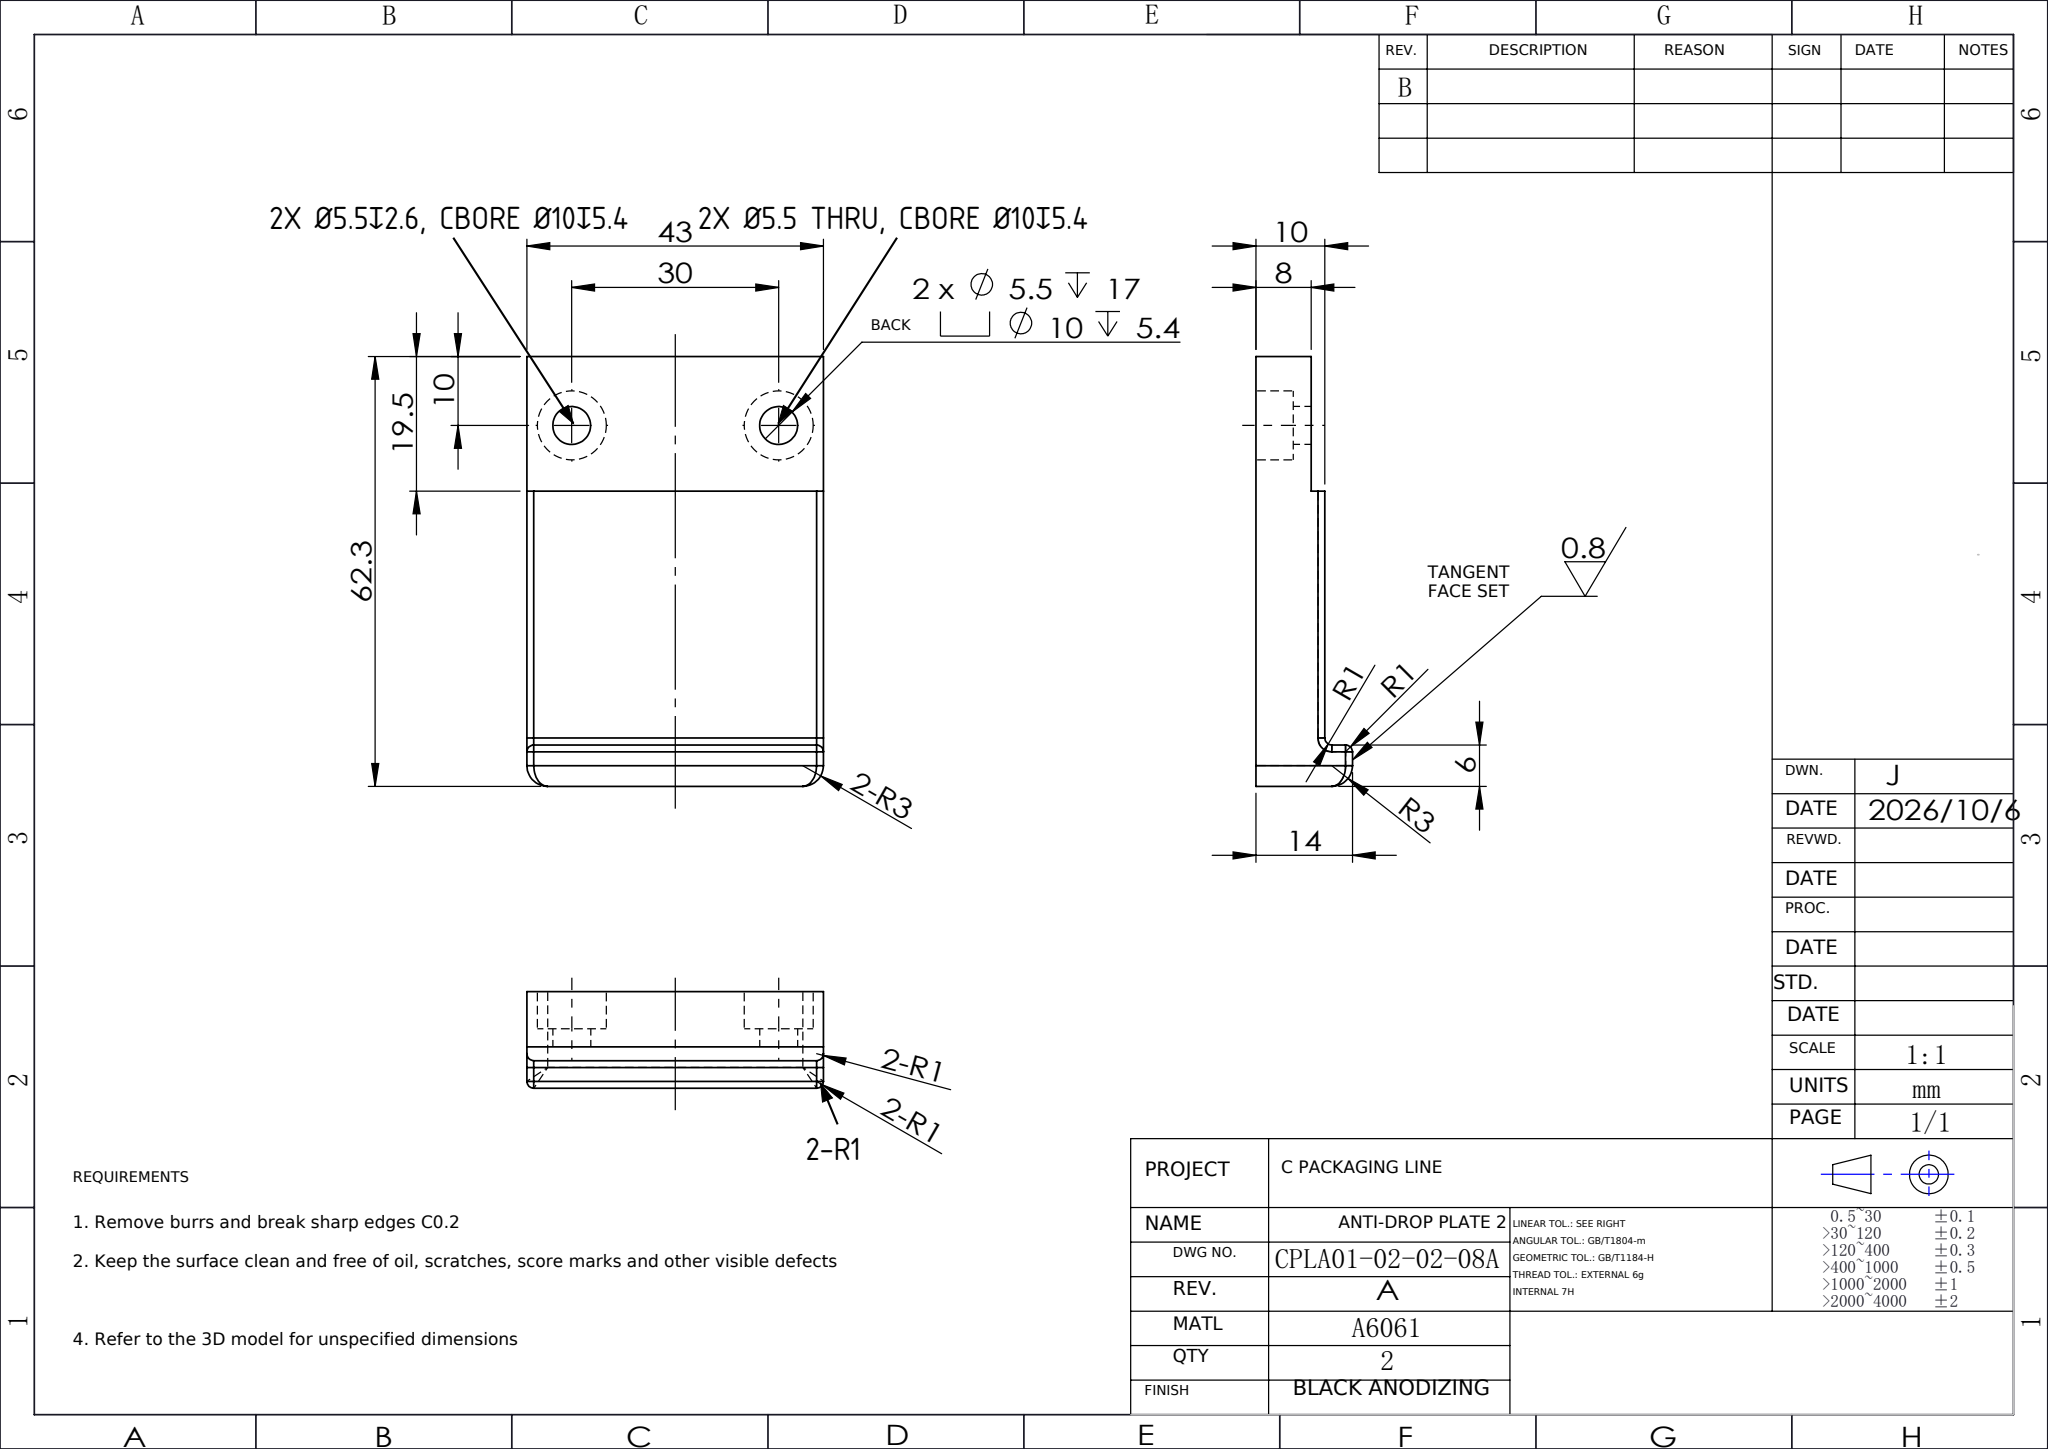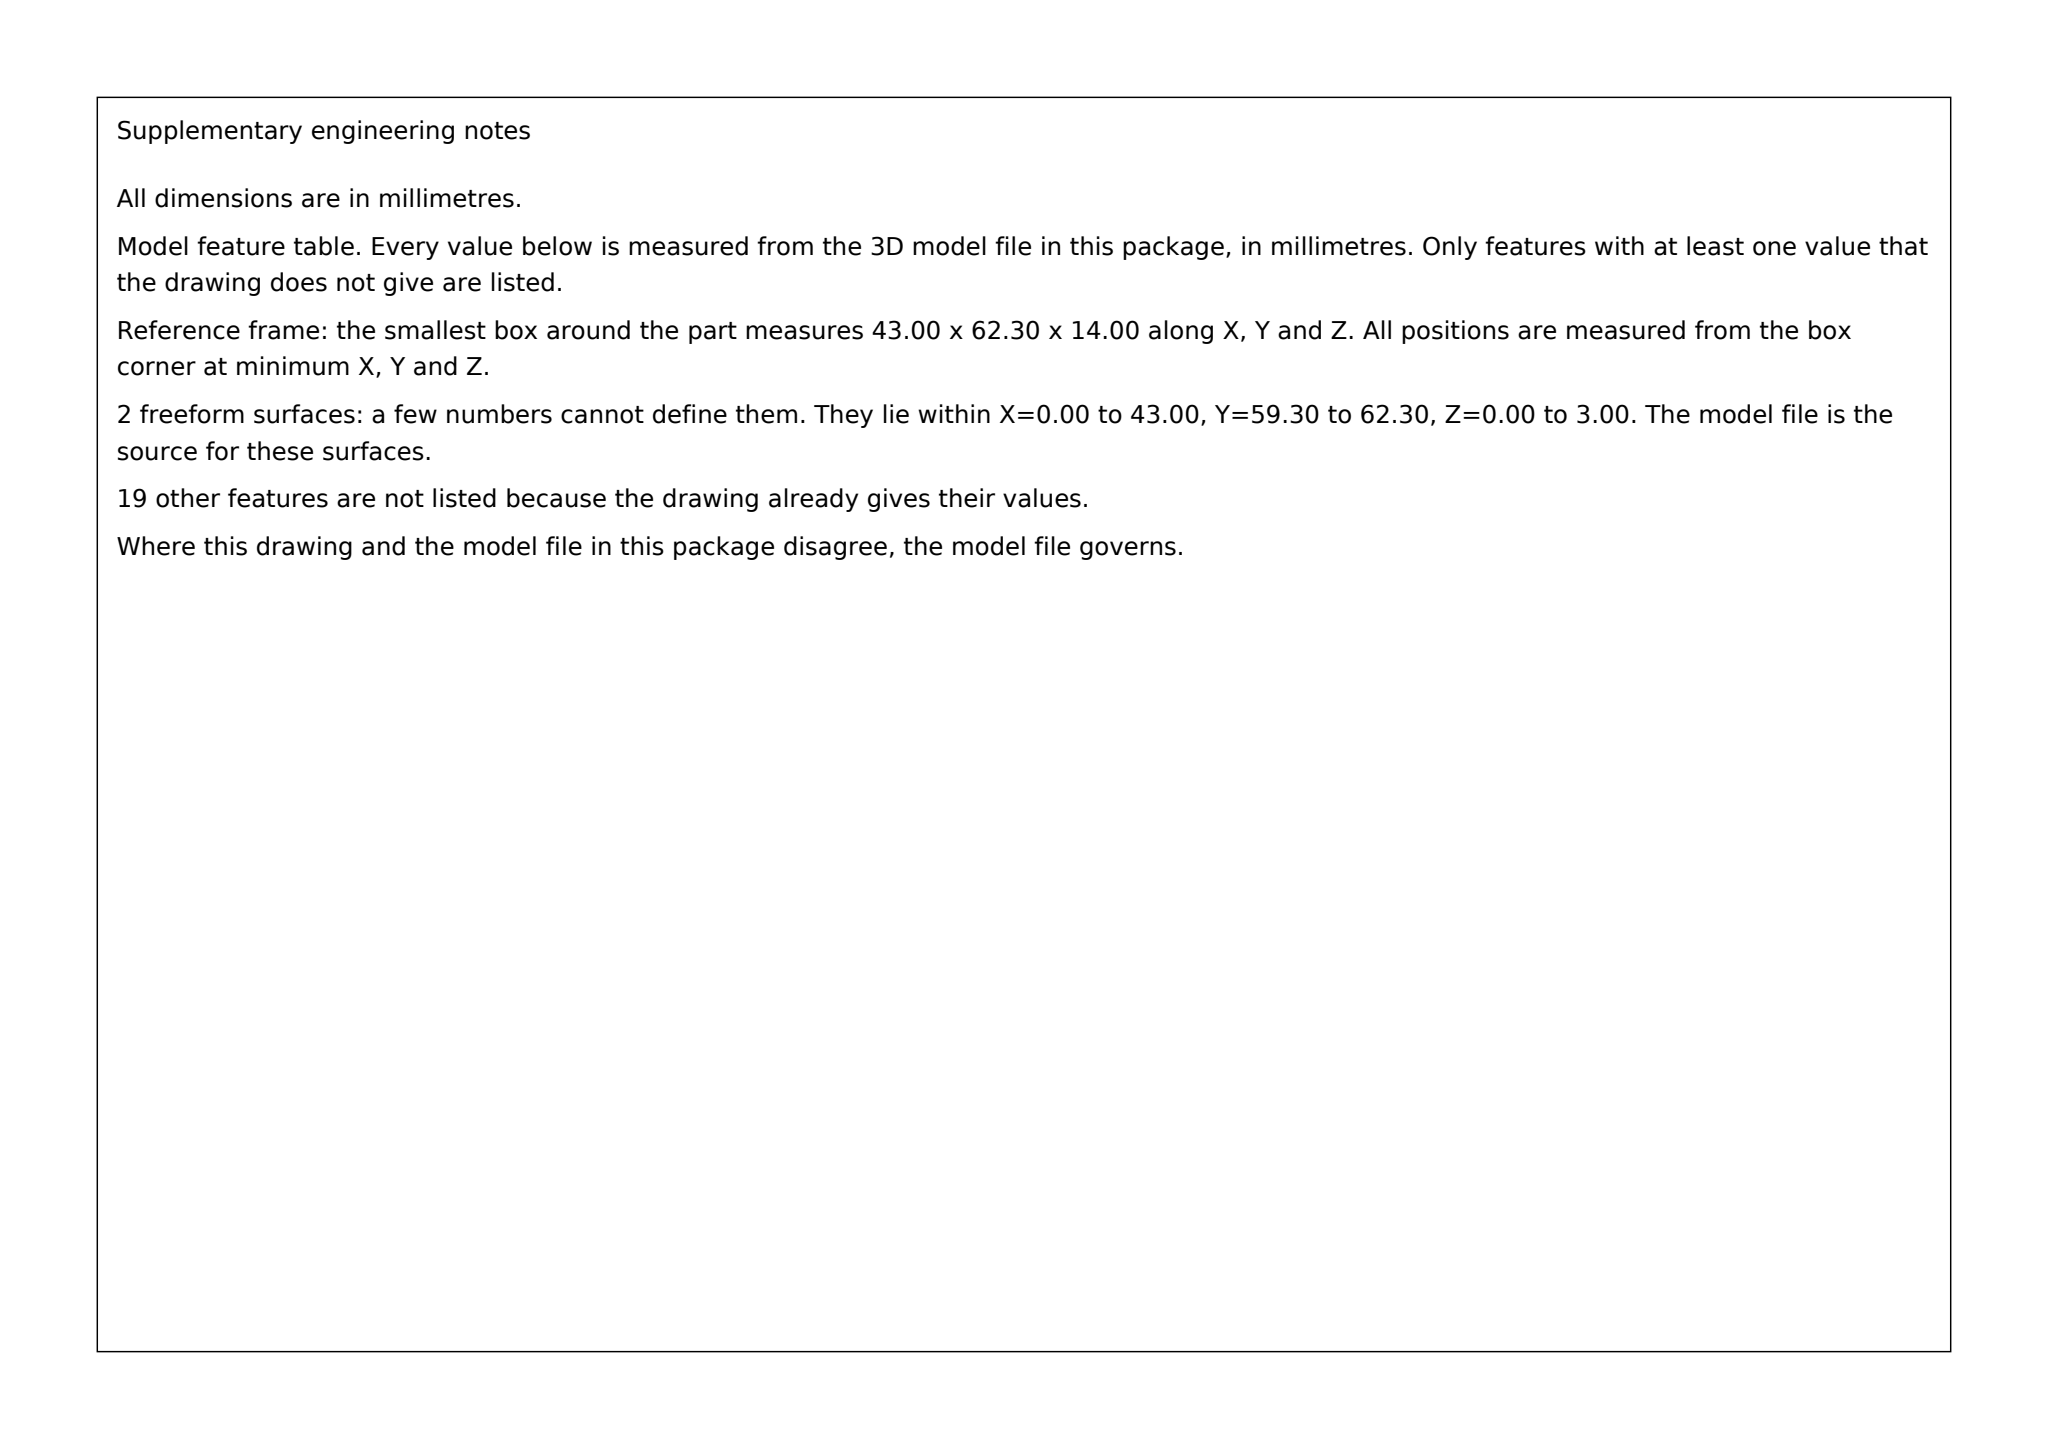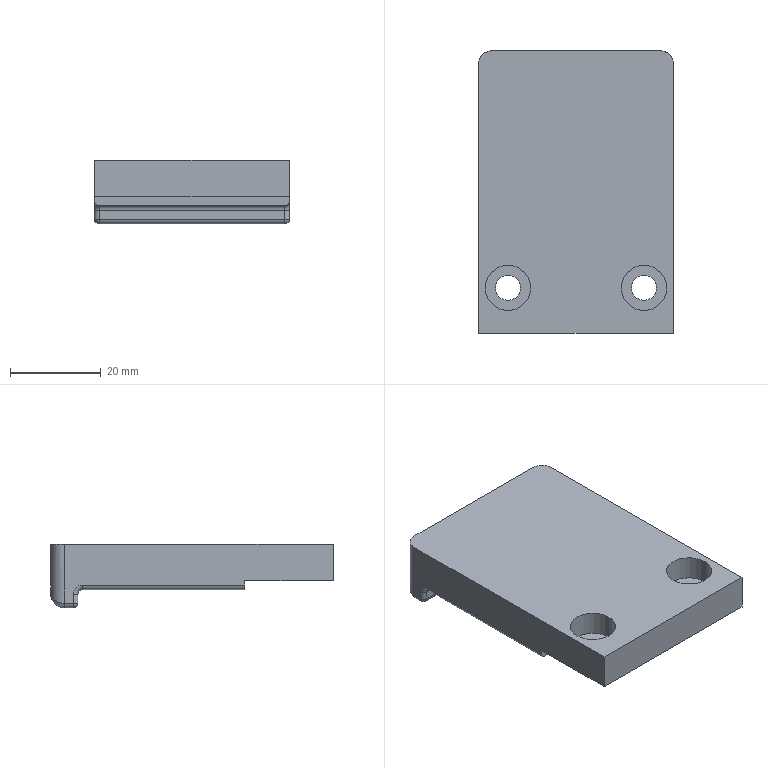Part | SolidWorks | mm | material A6061 | 1 solid | 37 faces | box 43 x 62.3 x 14 mm | volume 25021 mm3 | cylinder 19 | plane 12 | sphere 2 | torus 2 | spline 2 | commonest cylinder face diameters 2 x8 10 x4 5.5 x4 6 x3
Drawing notes:
2 x Ø5.5 THRU 8 TAB: HT 2.6, BACK C'BORE Ø10 HT 5.4 | from the solid: Ø5.5 bore z 6.0-8.6 (2.6 deep); Ø10 bore z 8.6-14.0 (5.4 deep); tab faces z=6.0 and z=14.0 (8 thick)
BOTTOM HOOK FOOT: 2-R1 VERT CORNER RNDS, R1 TORUS BLENDS | from the solid: Convex arcs dia 2.0 axis z at (x=1,y=57.3) and (x=42,y=57.3), z 1->3, 90 deg; tori minor_r 1.0 major 2.0 qty 2; side faces x=0/43 and face y=56.3 (x 1-42, z 1-3)
2 x Ø5.5 THRU (8 THK); BACK C'BORE Ø10 DP 5.4 - 17 VOID | from the solid: Bores Ø5.5 axis z at (6.5,10) and (36.5,10) from z=6.0 to 8.6; Ø10 c'bore same axes z=8.6 to 14.0 (5.4 deep from top face z=14); tab thickness z=6..14 = 8